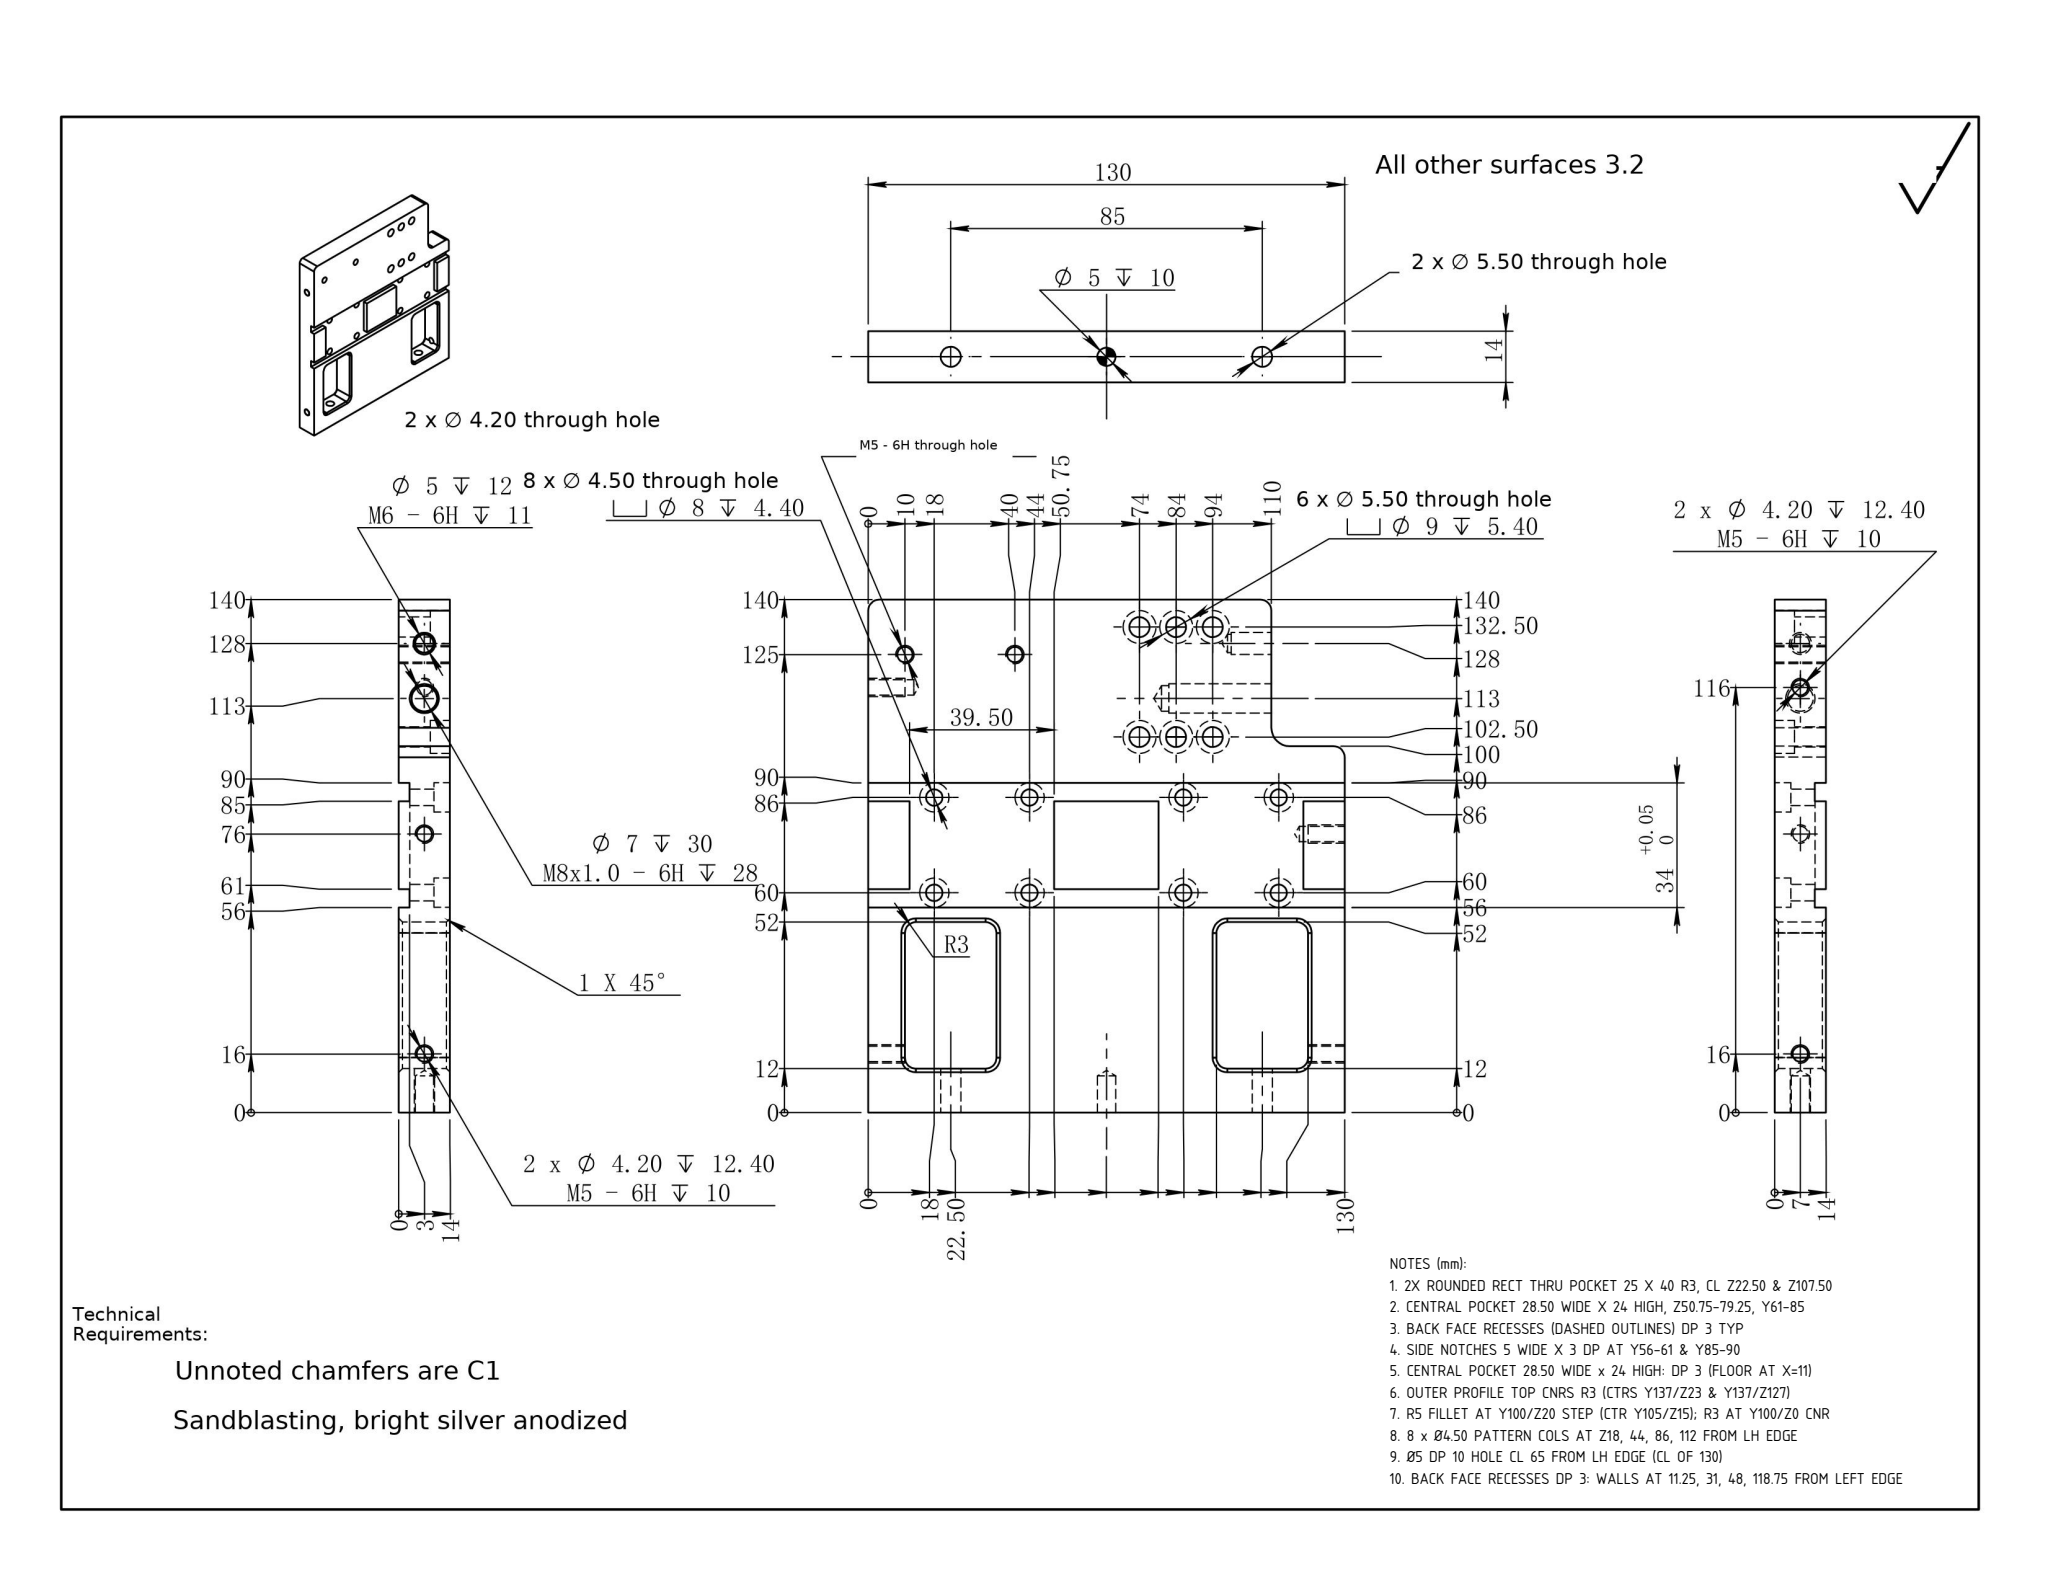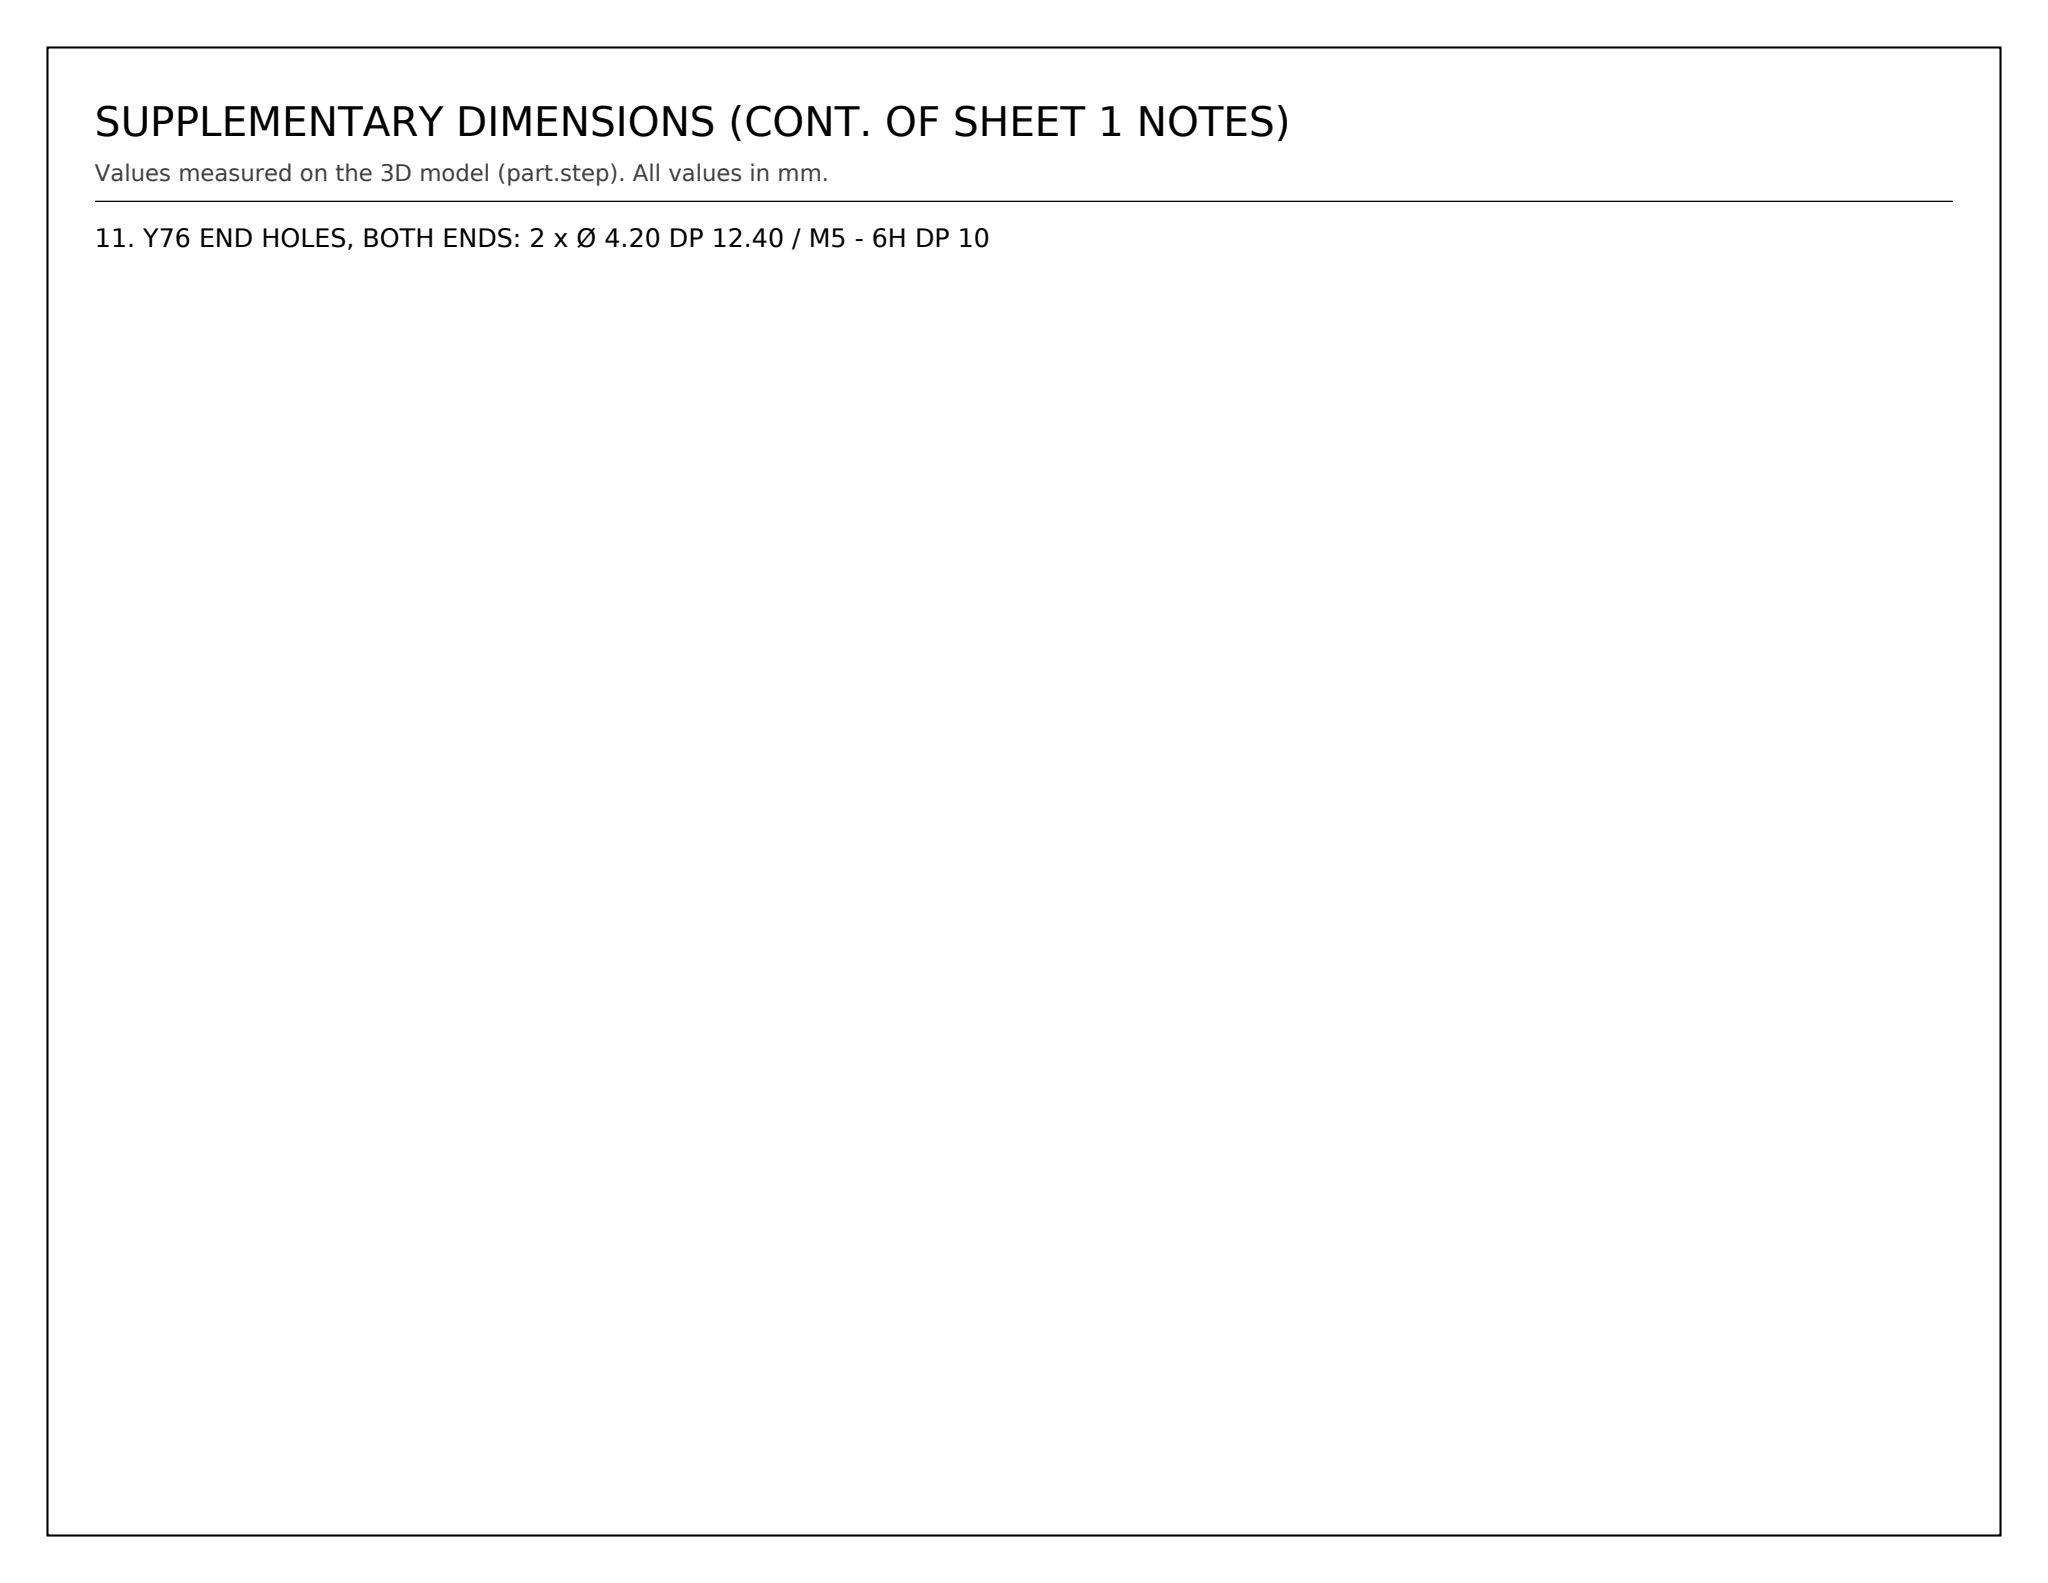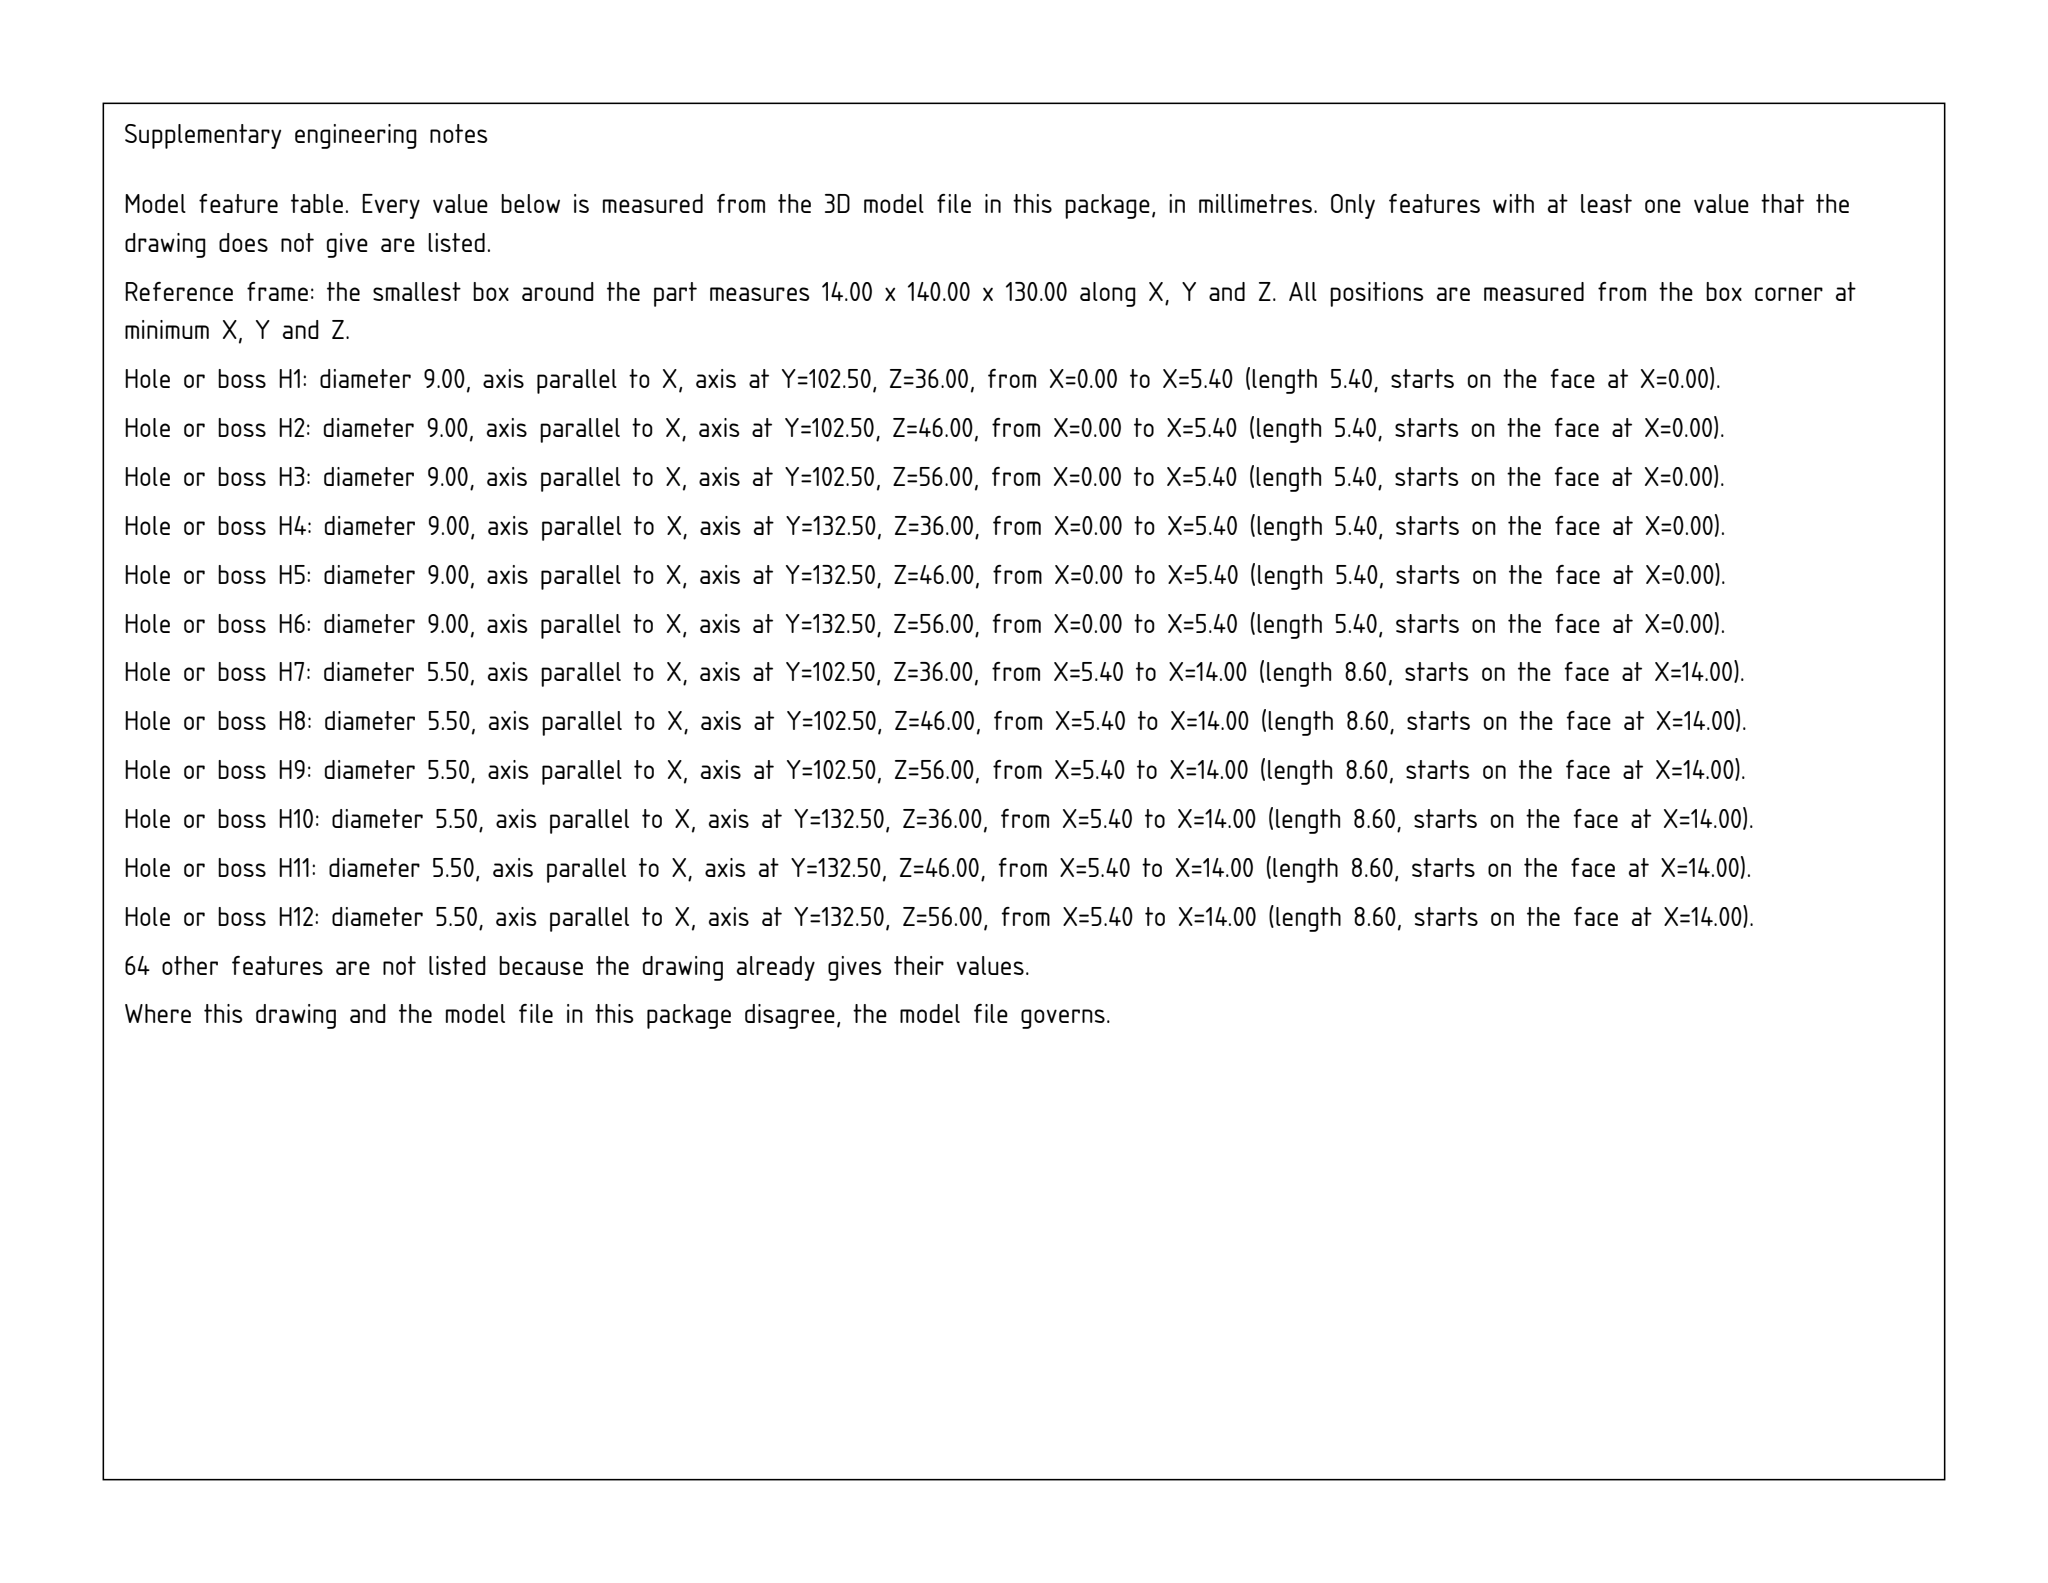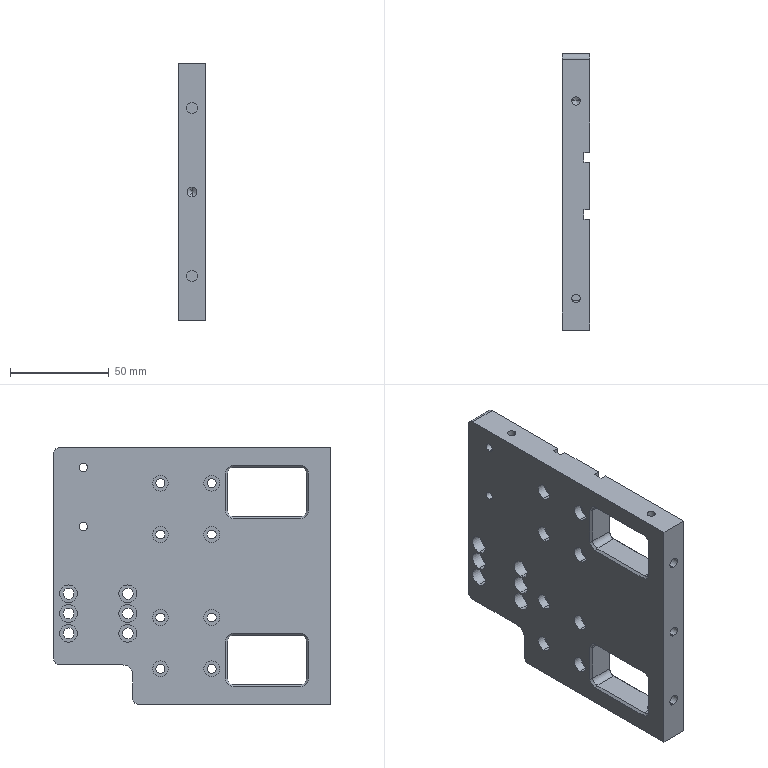Part | SolidWorks | mm | 1 solid | 185 faces | box 14 x 140 x 130 mm | volume 196423 mm3 | cylinder 94 | plane 65 | cone 26 | commonest cylinder face diameters 8 x18 5.5 x16 4.5 x16 6 x13 4.2 x12 9 x12 5 x4 7 x2
Drawing notes:
2X ROUNDED RECT THRU POCKET 25 X 40 R3, CL Z22.50 & Z107.50 | from the solid: z planes 10/35 & 95/120 = 25 wide, CL 22.5 & 107.5; y planes 12 & 52 = 40; thru 14 in X
CENTRAL POCKET 28.50 WIDE X 24 HIGH, Z50.75-79.25, Y61-85 | from the solid: z planes 50.75 & 79.25 = 28.50; y planes 61 & 85 = 24; centered on Ø5 hole at z=65
BACK FACE RECESSES (DASHED OUTLINES) DP 3 TYP | from the solid: single non-hole x plane at 11.0 vs 14.0 back face: 14-11 = 3 deep
SIDE NOTCHES 5 WIDE X 3 DP AT Y56-61 & Y85-90 | from the solid: y planes 56/61 and 85/90 = 5 wide; floor plane x=11.0 from x=14.0 face = 3 deep
CENTRAL POCKET 28.50 WIDE x 24 HIGH: DP 3 (FLOOR AT X=11) | from the solid: x-plane 11.0 (1 face) vs front face x=14; pocket Z50.75-79.25, Y61-85
OUTER PROFILE TOP CNRS R3 (CTRS Y137/Z23 & Y137/Z127) | from the solid: cyl dia6 x-axis at (y137,z23) & (y137,z127), len 14
R5 FILLET AT Y100/Z20 STEP (CTR Y105/Z15); R3 AT Y100/Z0 CNR | from the solid: cyl dia10 x-axis at (y105,z15) len 14; cyl dia6 x-axis at (y97,z3) len 14
8 x Ø4.50 PATTERN COLS AT Z18, 44, 86, 112 FROM LH EDGE | from the solid: dia4.5 x-axis holes at z=18,44,86,112 on y=60 and y=86
Ø5 DP 10 HOLE CL 65 FROM LH EDGE (CL OF 130) | from the solid: dia5 y-axis cyl at (x7, z65), len 10
BACK FACE RECESSES DP 3: WALLS AT 11.25, 31, 48, 118.75 FROM LEFT EDGE | from the solid: z-planes at 11.25, 31, 48, 118.75; recess floor x=3 (x-planes 0/14, depth 3 per left view 0-3-14)
Y76 END HOLES, BOTH ENDS: 2 x Ø 4.20 DP 12.40 / M5 - 6H DP 10 | from the solid: cylinders [4.2,'z',[7.0,76.0,null],12.4,2] - same size/depth as Y116 holes [4.2,'z',[7.0,116.0,null],12.4,2] called out M5-6H ↧10
build123d program:
from build123d import *

# Parameters (mm, degrees)
SKETCH1_W                                       = 14
SKETCH1_H                                       = 130
BOSS_EXTRUDE1_DEPTH                             = 140
SKETCH2_W                                       = 130
SKETCH2_H                                       = 34
CUT_EXTRUDE1_DEPTH                              = 3
SKETCH3_W                                       = 25
SKETCH3_H                                       = 40
CUT_EXTRUDE2_DEPTH                              = 155.987
F_5_5_5_5_DIAMETER_HOLE1_D                      = 5.5
F_5_5_5_5_DIAMETER_HOLE1_DEPTH                  = 12
FILLET1_R                                       = 3
CHAMFER1_SIZE                                   = 1
FILLET1_OF_MIRROR1_R                            = 3
CHAMFER1_OF_MIRROR1_SIZE                        = 1
F_5_0_5_DIAMETER_HOLE1_D                        = 5
F_5_0_5_DIAMETER_HOLE1_DEPTH                    = 10
F_5_0_5_DIAMETER_HOLE1_TIP                      = 1.502
SKETCH8_W                                       = 28.5
SKETCH8_H                                       = 24
SKETCH8_W_2                                     = 11.25
BOSS_EXTRUDE2_DEPTH                             = 3
M4_HEX_SOCKET_HEAD_CAP_SCREW_CBORE1_D           = 4.5
M4_HEX_SOCKET_HEAD_CAP_SCREW_CBORE1_CBORE_D     = 8
M4_HEX_SOCKET_HEAD_CAP_SCREW_CBORE1_CBORE_DEPTH = 4.4
M5_HEX_SOCKET_HEAD_CAP_SCREW_CBORE1_D           = 5.5
M5_HEX_SOCKET_HEAD_CAP_SCREW_CBORE1_CBORE_D     = 9
M5_HEX_SOCKET_HEAD_CAP_SCREW_CBORE1_CBORE_DEPTH = 5.4
LPATTERN1_COUNT                                 = 2
LPATTERN1_PITCH                                 = 10
LPATTERN1_COL_COUNT                             = 2
LPATTERN1_COL_PITCH                             = 10
SKETCH15_W                                      = 20
SKETCH15_H                                      = 40
CUT_EXTRUDE3_DEPTH                              = 155.987
FILLET2_R                                       = 3
FILLET3_R                                       = 5
M8X1_0_TAPPED_HOLE1_D                           = 7
M8X1_0_TAPPED_HOLE1_DEPTH                       = 30
M8X1_0_TAPPED_HOLE1_CBORE_D                     = 8
M8X1_0_TAPPED_HOLE1_CBORE_DEPTH                 = 28
M8X1_0_TAPPED_HOLE1_TIP                         = 2.103
M6_TAPPED_HOLE1_D                               = 5
M6_TAPPED_HOLE1_DEPTH                           = 12
M6_TAPPED_HOLE1_CBORE_D                         = 6
M6_TAPPED_HOLE1_CBORE_DEPTH                     = 11
M6_TAPPED_HOLE1_TIP                             = 1.502
M5_TAPPED_HOLE1_D                               = 4.2
M5_TAPPED_HOLE2_D                               = 4.2
M5_TAPPED_HOLE2_DEPTH                           = 12.4
M5_TAPPED_HOLE2_TIP                             = 1.262
M5_TAPPED_HOLE3_D                               = 4.2
M5_TAPPED_HOLE3_DEPTH                           = 12.4
M5_TAPPED_HOLE3_TIP                             = 1.262


with BuildPart() as part:
    # Sketch1 → Boss-Extrude1 (new body)
    with BuildSketch(Plane(origin=(0, 0, 0), x_dir=(1, 0, 0), z_dir=(0, 1, 0))):
        Rectangle(SKETCH1_W, SKETCH1_H)
    extrude(amount=BOSS_EXTRUDE1_DEPTH)

    # Sketch2 → Cut-Extrude1 (cut)
    with BuildSketch(Plane(origin=(7, 0, 0), x_dir=(0, 0, -1), z_dir=(1, 0, 0))):
        with Locations((0, 73)):
            Rectangle(SKETCH2_W, SKETCH2_H)
    extrude(amount=-CUT_EXTRUDE1_DEPTH, mode=Mode.SUBTRACT)

    # Sketch3 → Cut-Extrude2 (cut, through all)
    with BuildSketch(Plane.ZY.offset(7)):
        with Locations((-42.5, 32)):
            Rectangle(SKETCH3_W, SKETCH3_H)
    cut_extrude2 = extrude(amount=-CUT_EXTRUDE2_DEPTH, mode=Mode.SUBTRACT)

    # 5.5 _5.5_ Diameter Hole1
    with Locations(Plane(origin=(0, 12, 0), x_dir=(1, 0, 0), z_dir=(0, 1, 0))):
        with Locations((0, 42.5)):
            f_5_5_5_5_diameter_hole1 = Hole(F_5_5_5_5_DIAMETER_HOLE1_D / 2, depth=F_5_5_5_5_DIAMETER_HOLE1_DEPTH)

    # Fillet1
    fillet1_edges = [part.edges().sort_by_distance(p)[0] for p in [
        (0, 52, -30),
        (0, 12, -30),
        (0, 12, -55),
        (0, 52, -55),
    ]]
    fillet(fillet1_edges, radius=FILLET1_R)

    # Chamfer1
    chamfer1_edges = [part.edges().sort_by_distance(p)[0] for p in [
        (-7, 32, -30),
        (7, 32, -30),
        (-7, 12, -42.5),
        (7, 12, -42.5),
        (-7, 32, -55),
        (7, 32, -55),
        (-7, 52, -42.5),
        (7, 52, -42.5),
        (-7, 12.879, -30.879),
        (7, 12.879, -30.879),
        (-7, 12.879, -54.121),
        (7, 12.879, -54.121),
        (-7, 51.121, -54.121),
        (7, 51.121, -54.121),
        (-7, 51.121, -30.879),
        (7, 51.121, -30.879),
    ]]
    chamfer(chamfer1_edges, length=CHAMFER1_SIZE)

    # Mirror1: Cut-Extrude2, 5.5 _5.5_ Diameter Hole1 across plane
    add(cut_extrude2.mirror(Plane.XY), mode=Mode.SUBTRACT)
    add(f_5_5_5_5_diameter_hole1.mirror(Plane.XY), mode=Mode.SUBTRACT)

    # Fillet1 of Mirror1
    fillet1_of_mirror1_edges = [part.edges().sort_by_distance(p)[0] for p in [
        (0, 52, 30),
        (0, 12, 30),
        (0, 12, 55),
        (0, 52, 55),
    ]]
    fillet(fillet1_of_mirror1_edges, radius=FILLET1_OF_MIRROR1_R)

    # Chamfer1 of Mirror1
    chamfer1_of_mirror1_edges = [part.edges().sort_by_distance(p)[0] for p in [
        (-7, 32, 30),
        (7, 32, 30),
        (-7, 12, 42.5),
        (7, 12, 42.5),
        (-7, 32, 55),
        (7, 32, 55),
        (-7, 52, 42.5),
        (7, 52, 42.5),
        (-7, 12.879, 30.879),
        (7, 12.879, 30.879),
        (-7, 12.879, 54.121),
        (7, 12.879, 54.121),
        (-7, 51.121, 54.121),
        (7, 51.121, 54.121),
        (-7, 51.121, 30.879),
        (7, 51.121, 30.879),
    ]]
    chamfer(chamfer1_of_mirror1_edges, length=CHAMFER1_OF_MIRROR1_SIZE)

    # 5.0 _5_ Diameter Hole1
    with Locations(Plane(origin=(0, 0, 0), x_dir=(-1, 0, 0), z_dir=(0, -1, 0))):
        with Locations((0, 0)):
            Hole(F_5_0_5_DIAMETER_HOLE1_D / 2, depth=F_5_0_5_DIAMETER_HOLE1_DEPTH)
            with Locations((0, 0, -(F_5_0_5_DIAMETER_HOLE1_DEPTH + F_5_0_5_DIAMETER_HOLE1_TIP / 2))):  # 118° drill point
                Cone(0, F_5_0_5_DIAMETER_HOLE1_D / 2, F_5_0_5_DIAMETER_HOLE1_TIP, mode=Mode.SUBTRACT)

    # Sketch8 → Boss-Extrude2 (add)
    with BuildSketch(Plane(origin=(4, 0, 0), x_dir=(0, 0, -1), z_dir=(1, 0, 0))):
        with Locations((0, 73)):
            Rectangle(SKETCH8_W, SKETCH8_H)
        with Locations((59.375, 73)):
            Rectangle(SKETCH8_W_2, SKETCH8_H)
        with Locations((-59.375, 73)):
            Rectangle(SKETCH8_W_2, SKETCH8_H)
    extrude(amount=BOSS_EXTRUDE2_DEPTH)

    # M4 Hex Socket Head Cap Screw CBORE1 (through all)
    with Locations(Plane.ZY.offset(7)):
        with Locations((-47, 86), (-21, 86), (-21, 60), (-47, 60), (21, 60), (21, 86), (47, 86), (47, 60)):
            CounterBoreHole(M4_HEX_SOCKET_HEAD_CAP_SCREW_CBORE1_D / 2, M4_HEX_SOCKET_HEAD_CAP_SCREW_CBORE1_CBORE_D / 2, M4_HEX_SOCKET_HEAD_CAP_SCREW_CBORE1_CBORE_DEPTH)

    # M5 Hex Socket Head Cap Screw CBORE1 (through all)
    with Locations(Plane.ZY.offset(7)):
        with Locations((-19, 132.5), (-19, 102.5)):
            m5_hex_socket_head_cap_screw_cbore1 = CounterBoreHole(M5_HEX_SOCKET_HEAD_CAP_SCREW_CBORE1_D / 2, M5_HEX_SOCKET_HEAD_CAP_SCREW_CBORE1_CBORE_D / 2, M5_HEX_SOCKET_HEAD_CAP_SCREW_CBORE1_CBORE_DEPTH)

    # LPattern1: M5 Hex Socket Head Cap Screw CBORE1 ×2
    with Locations(*[(0, 0, i * LPATTERN1_PITCH) for i in range(1, LPATTERN1_COUNT)]):
        add(m5_hex_socket_head_cap_screw_cbore1, mode=Mode.SUBTRACT)

    # LPattern1 col: M5 Hex Socket Head Cap Screw CBORE1 ×2
    with Locations(*[(0, 0, -i * LPATTERN1_COL_PITCH) for i in range(1, LPATTERN1_COL_COUNT)]):
        add(m5_hex_socket_head_cap_screw_cbore1, mode=Mode.SUBTRACT)

    # Sketch15 → Cut-Extrude3 (cut, through all)
    with BuildSketch(Plane(origin=(7, 0, 0), x_dir=(0, 0, -1), z_dir=(1, 0, 0))):
        with Locations((55, 120)):
            Rectangle(SKETCH15_W, SKETCH15_H)
    extrude(amount=-CUT_EXTRUDE3_DEPTH, mode=Mode.SUBTRACT)

    # Fillet2
    fillet2_edges = [part.edges().sort_by_distance(p)[0] for p in [
        (0, 140, 65),
        (0, 100, -65),
        (0, 140, -45),
    ]]
    fillet(fillet2_edges, radius=FILLET2_R)

    # Fillet3
    fillet3_edges = [part.edges().sort_by_distance(p)[0] for p in [
        (0, 100, -45),
    ]]
    fillet(fillet3_edges, radius=FILLET3_R)

    # M8x1.0 Tapped Hole1
    with Locations(Plane(origin=(0, 0, -45), x_dir=(-1, 0, 0), z_dir=(0, 0, -1))):
        with Locations((0, 113)):
            CounterBoreHole(M8X1_0_TAPPED_HOLE1_D / 2, M8X1_0_TAPPED_HOLE1_CBORE_D / 2, M8X1_0_TAPPED_HOLE1_CBORE_DEPTH, depth=M8X1_0_TAPPED_HOLE1_DEPTH)
            with Locations((0, 0, -(M8X1_0_TAPPED_HOLE1_DEPTH + M8X1_0_TAPPED_HOLE1_TIP / 2))):  # 118° drill point
                Cone(0, M8X1_0_TAPPED_HOLE1_D / 2, M8X1_0_TAPPED_HOLE1_TIP, mode=Mode.SUBTRACT)

    # M6 Tapped Hole1
    with Locations(Plane(origin=(0, 0, -45), x_dir=(-1, 0, 0), z_dir=(0, 0, -1))):
        with Locations((0, 128)):
            CounterBoreHole(M6_TAPPED_HOLE1_D / 2, M6_TAPPED_HOLE1_CBORE_D / 2, M6_TAPPED_HOLE1_CBORE_DEPTH, depth=M6_TAPPED_HOLE1_DEPTH)
            with Locations((0, 0, -(M6_TAPPED_HOLE1_DEPTH + M6_TAPPED_HOLE1_TIP / 2))):  # 118° drill point
                Cone(0, M6_TAPPED_HOLE1_D / 2, M6_TAPPED_HOLE1_TIP, mode=Mode.SUBTRACT)

    # M5 Tapped Hole1 (through all)
    with Locations(Plane.ZY.offset(7)):
        with Locations((25, 125), (55, 125)):
            Hole(M5_TAPPED_HOLE1_D / 2)

    # M5 Tapped Hole2
    with Locations(Plane(origin=(0, 0, -65), x_dir=(-1, 0, 0), z_dir=(0, 0, -1))):
        with Locations((0, 16), (0, 76)):
            Hole(M5_TAPPED_HOLE2_D / 2, depth=M5_TAPPED_HOLE2_DEPTH)
            with Locations((0, 0, -(M5_TAPPED_HOLE2_DEPTH + M5_TAPPED_HOLE2_TIP / 2))):  # 118° drill point
                Cone(0, M5_TAPPED_HOLE2_D / 2, M5_TAPPED_HOLE2_TIP, mode=Mode.SUBTRACT)

    # M5 Tapped Hole3
    with Locations(Plane.XY.offset(65)):
        with Locations((0, 116), (0, 16)):
            Hole(M5_TAPPED_HOLE3_D / 2, depth=M5_TAPPED_HOLE3_DEPTH)
            with Locations((0, 0, -(M5_TAPPED_HOLE3_DEPTH + M5_TAPPED_HOLE3_TIP / 2))):  # 118° drill point
                Cone(0, M5_TAPPED_HOLE3_D / 2, M5_TAPPED_HOLE3_TIP, mode=Mode.SUBTRACT)


solid = part.part